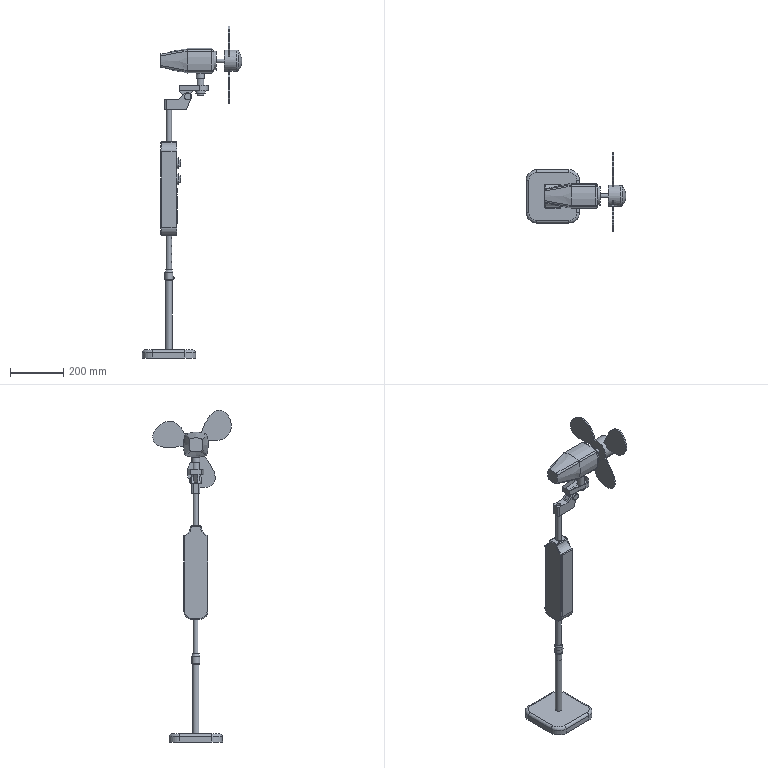Assembly | NX | mm | 16 component files | 24 solids | 428 faces | box 373.05 x 294.07 x 1244.69 mm | volume 3476377 mm3 | plane 214 | cylinder 147 | torus 29 | spline 13 | sphere 12 | other 7 | cone 6 | commonest cylinder face diameters 6 x37 20 x12 5 x12 15 x10 30 x9 25 x9 10 x6 8 x5
Bill of materials:
unnamed part 1 | 1 |  | Thin hexagonal prism with a large central circular through-bore; nut-like shape, low height relative to across-flats width.
unnamed part 2 | 1 |  | Block-shaped bracket. One end is a flat tab with rounded corners and a vertical through-hole. The other end is a raised clevis with two parallel lugs that have rounded ends and coaxial cross holes, separated by an open slot. The body has an angled side profile.
unnamed part 3 | 1 |  | Three-bladed propeller- or fan-like rotor: a short cylindrical hub with one domed end and three thin, rounded, lobe-shaped blades spaced evenly around it.
unnamed part 4 | 1 |  | Elongated block with a rounded-rectangle cross-section and a fully rounded bottom end. The top narrows through concave fillets into a neck with a small hole in its top face. One broad face has two circular recessed features with small central holes and a shallow outlined recessed panel.
unnamed part 5 | 1 |  | Cylindrical sleeve with tapered or chamfered conical ends and a large axial through-bore. A small radial tubular boss with its own hole sticks out from the outer wall near one end.
unnamed part 6 | 1 |  | Headed cylindrical pin: a plain, straight cylindrical shank with a short, larger-diameter flat disc head at one end.
unnamed part 7 | 1 |  | Long, thin-walled straight round tube with one small radial hole through the wall near one end.
unnamed part 8 | 1 |  | Plain, long, thin-walled straight round tube with open ends and no other visible features.
unnamed part 9 | 1 |  | Elongated body with a rounded-square cross-section. It tapers along part of its length toward one end; the larger end is flat with a short round boss and a thin cylindrical rod sticking out along the axis. A larger cylindrical protrusion also appears to extend sideways from the body in two views.
unnamed part 10 | 1 |  | Thin flat plate with one semicircular rounded end and rounded corners at the other. One face carries two columns of raised features: four small round bosses and four larger oval raised pads.
unnamed part 11 | 1 |  | Solid cylindrical shaft with an integral straight-toothed spur-gear or pinion section at one end. The toothed section has a larger outside diameter than the shaft.
unnamed part 12 | 1 |  | Long, thin-walled straight round tube with a row of six small, evenly spaced radial holes along one side.
unnamed part 13 | 1 |  | Tapered, open-top tray-like arm with a thin perimeter wall around a shallow pocket. One end is wide and squared; the other end is narrow and rounded. A vertical hollow cylindrical tube passes through the rounded end. It sticks out well above the wall and below the base, and has stepped diameters below. A triangular lug with a transverse round hole hangs below the base.
unnamed part 14 | 1 |  | Thin, square, plate-like block with large-radius rounded corners and a filleted or rounded top perimeter edge. There is a small round hole in the center of the top face.
unnamed part 15 | 2 |  | Circular disc with rounded perimeter edges. One flat face has a single raised, elongated rib with rounded ends running along a diameter. Seen from the side, the rib has a concave (inwardly curved) outer edge and rounded corners.
Mates:
1. fix | base 1 component
2. concentric | base 1 edge | support_rod_3 1 edge
3. concentric | lock_sleeve 1 edge | support_rod_3 1 edge
4. align lock | support_rod_2 1 face | support_rod_3 1 face
5. align lock | support_rod_2 1 face | lock_sleeve 1 face
6. concentric | lock_sleeve 1 edge | locking_knob 1 edge
7. concentric | housing 1 edge | support_rod_2 1 edge
8. parallel | housing 1 face | base 1 face
9. concentric | housing 1 edge | knob 2 edge
10. touch align | control_panel 1 face | housing 1 face
11. touch align | control_panel 1 face | housing 1 face
12. touch align | control_panel 1 face | housing 1 face
13. concentric | housing 1 edge | support_rod_1 1 edge
14. concentric | up_down_bracket 1 edge | support_rod_1 1 edge
15. parallel | up_down_bracket 1 face | base 1 face
16. concentric | left_right_bracket 1 edge | up_down_bracket 1 edge
17. concentric | up_down_bracket 1 edge | bolt 1 arc
18. concentric | nut 1 arc | up_down_bracket 1 edge
19. concentric | left_right_bracket 1 edge | motor 1 edge
20. concentric | motor 1 edge | fan_blade 1 edge
21. concentric | knob 1 edge | housing 1 edge